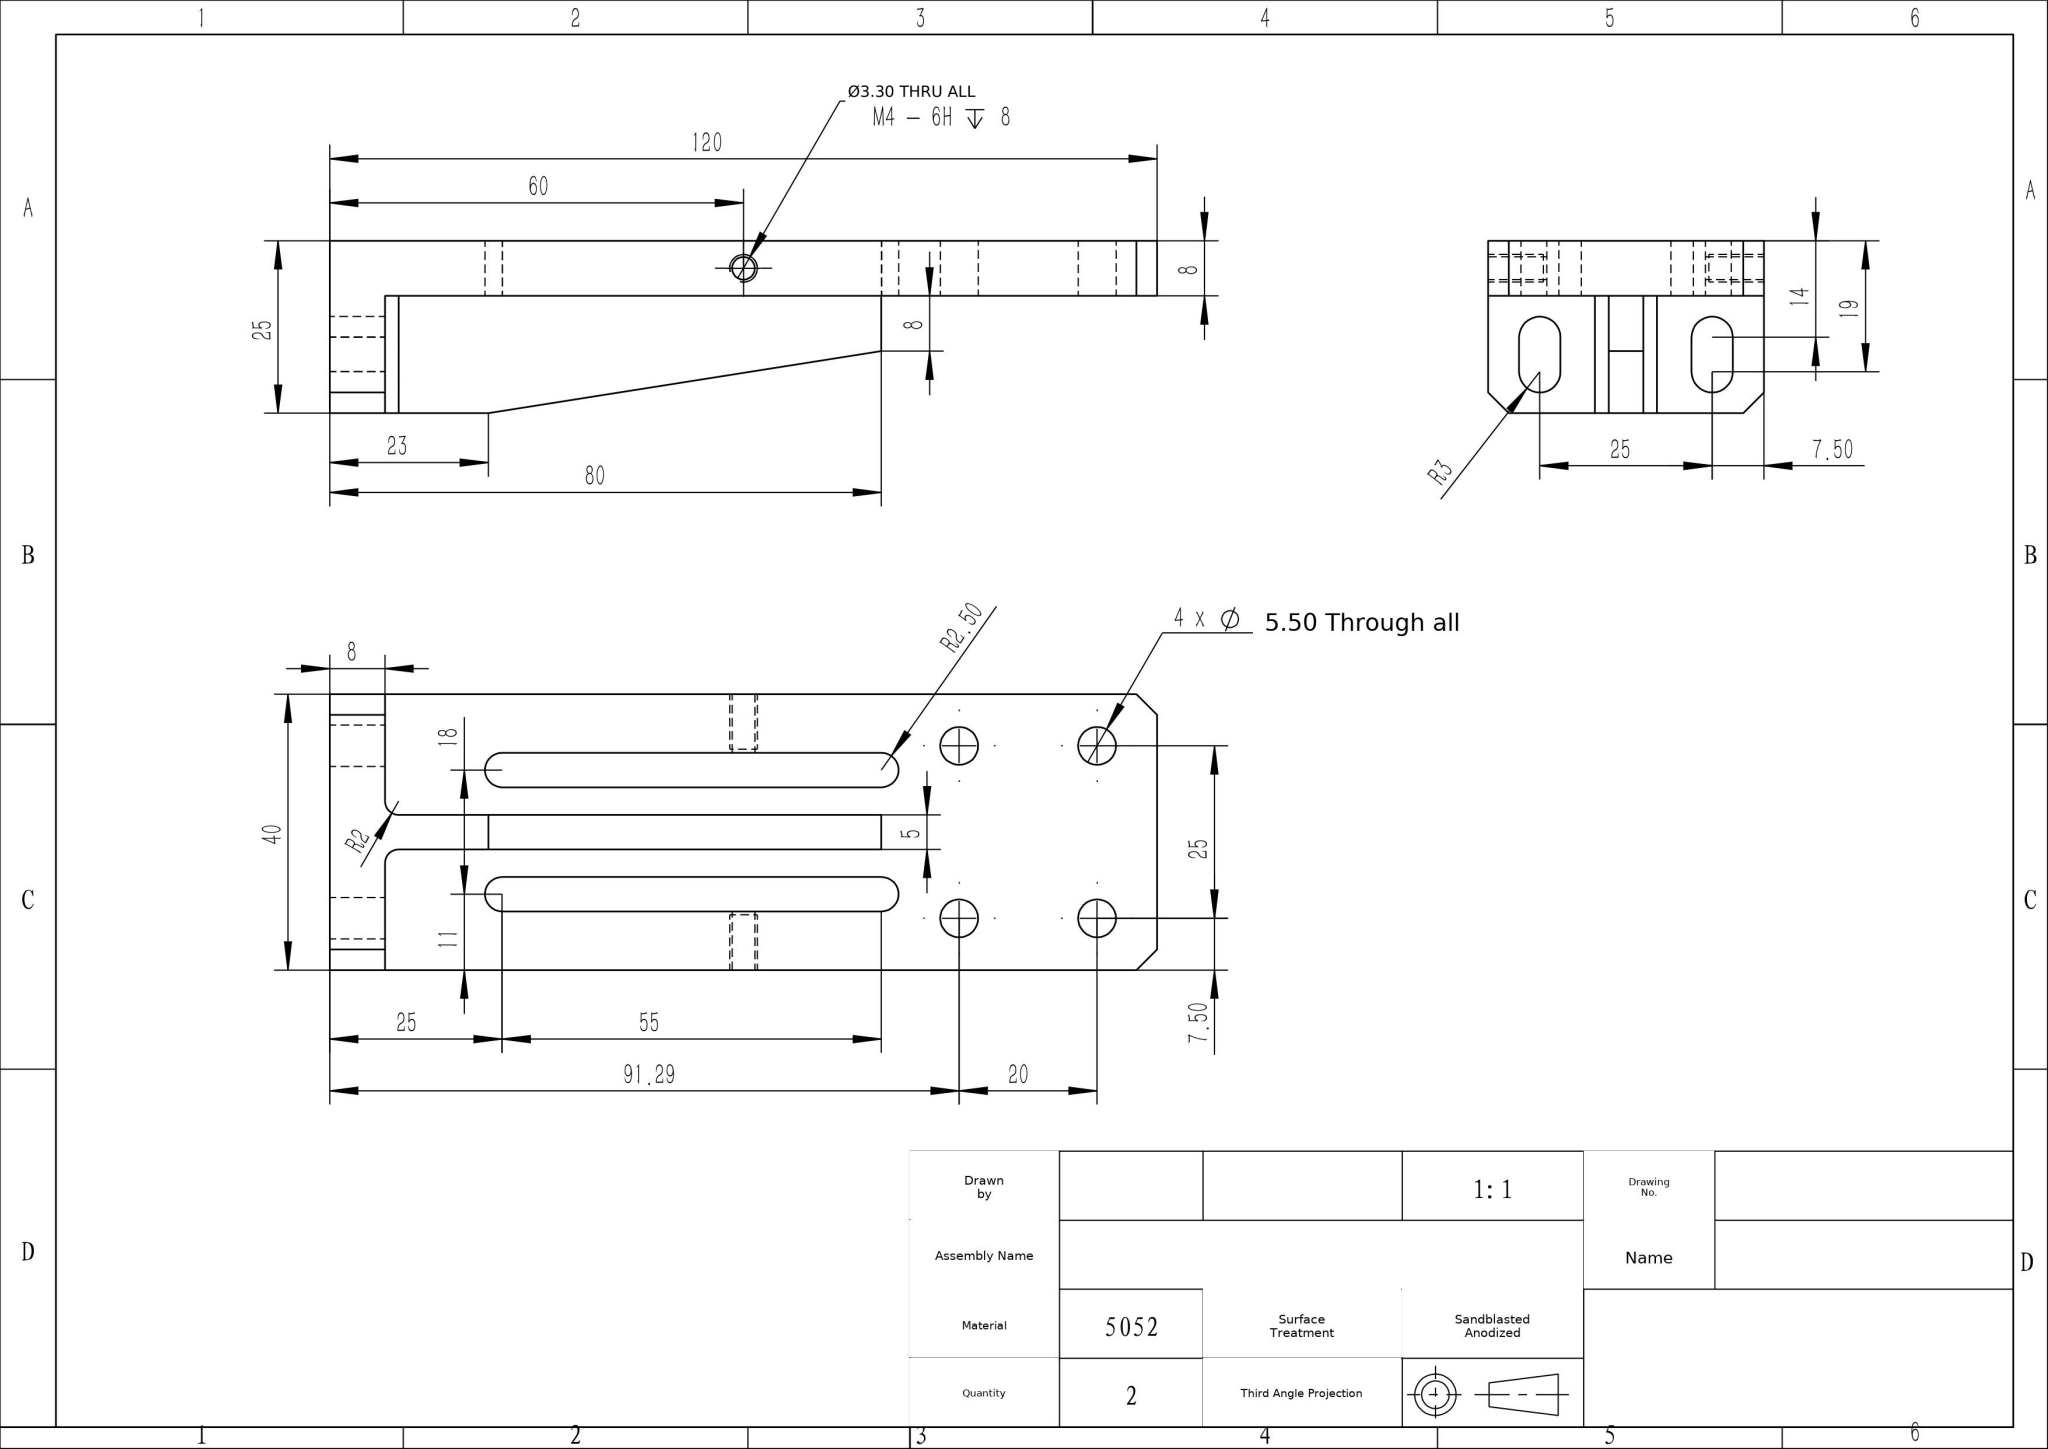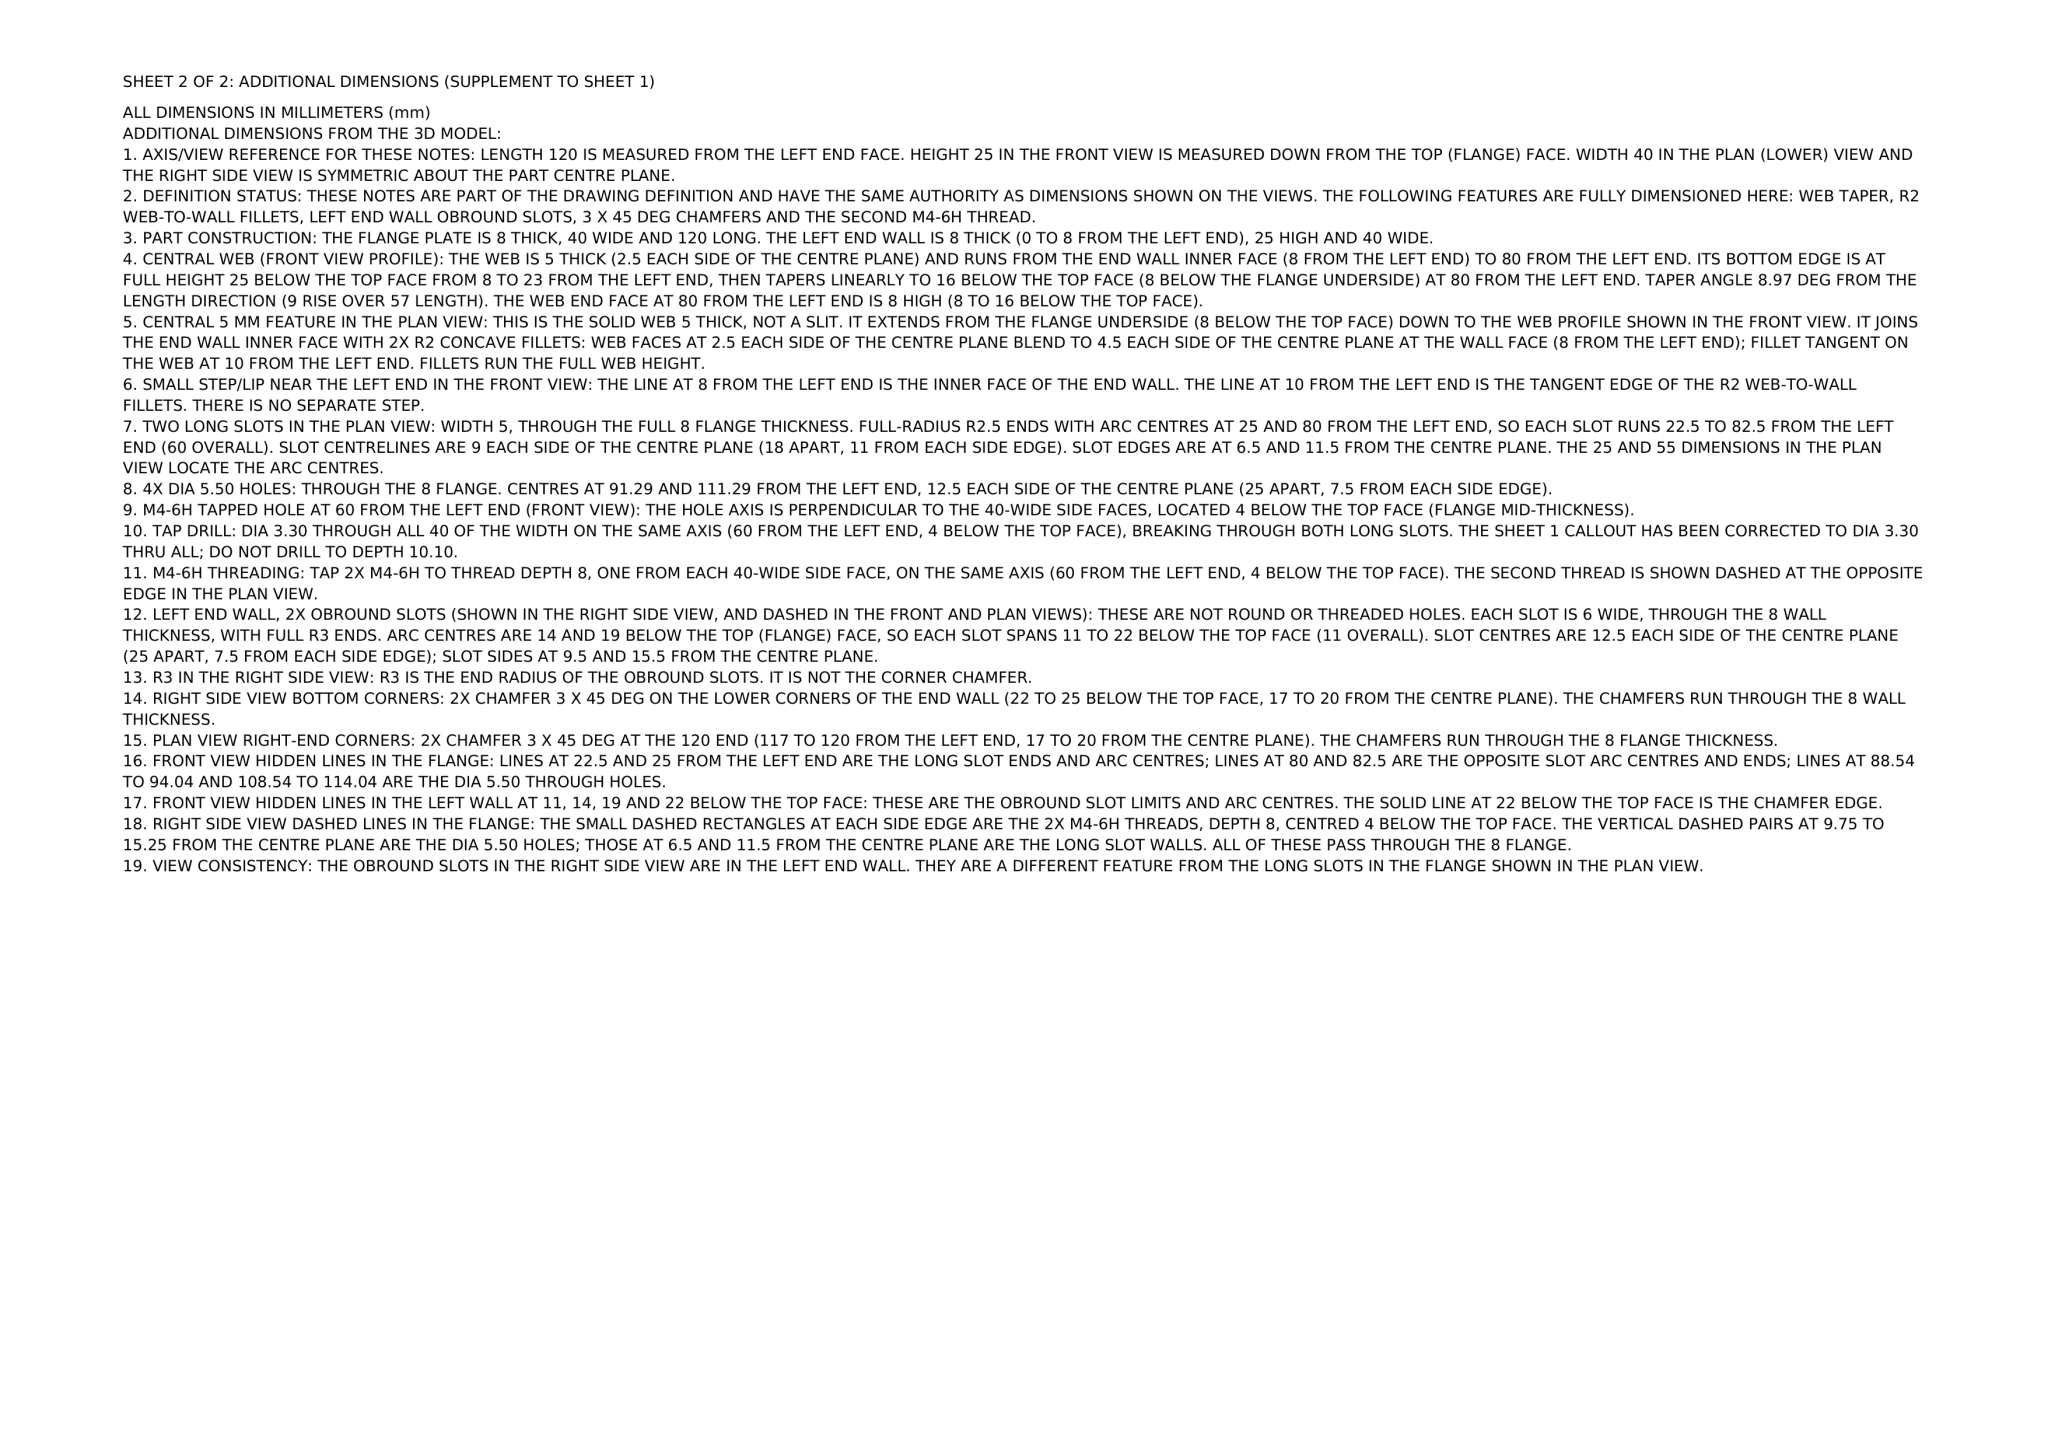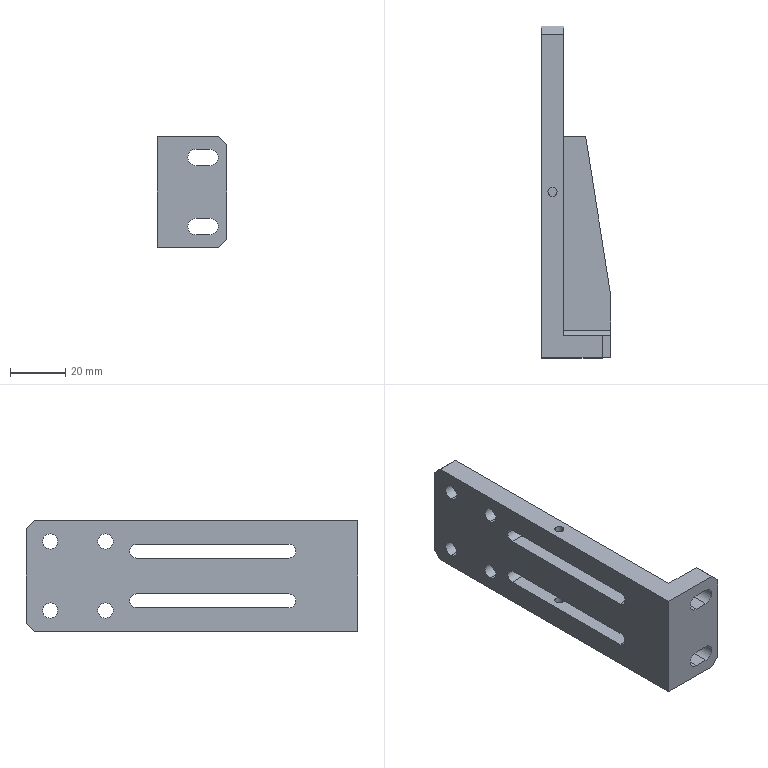Part | NX | mm | Slotted L-Shaped Wall Bracket | 1 solid | 51 faces | box 25 x 120 x 40 mm | volume 42010 mm3 | cylinder 26 | plane 25 | commonest cylinder face diameters 5.5 x8 5 x6 6 x6 3.3 x4 4 x2